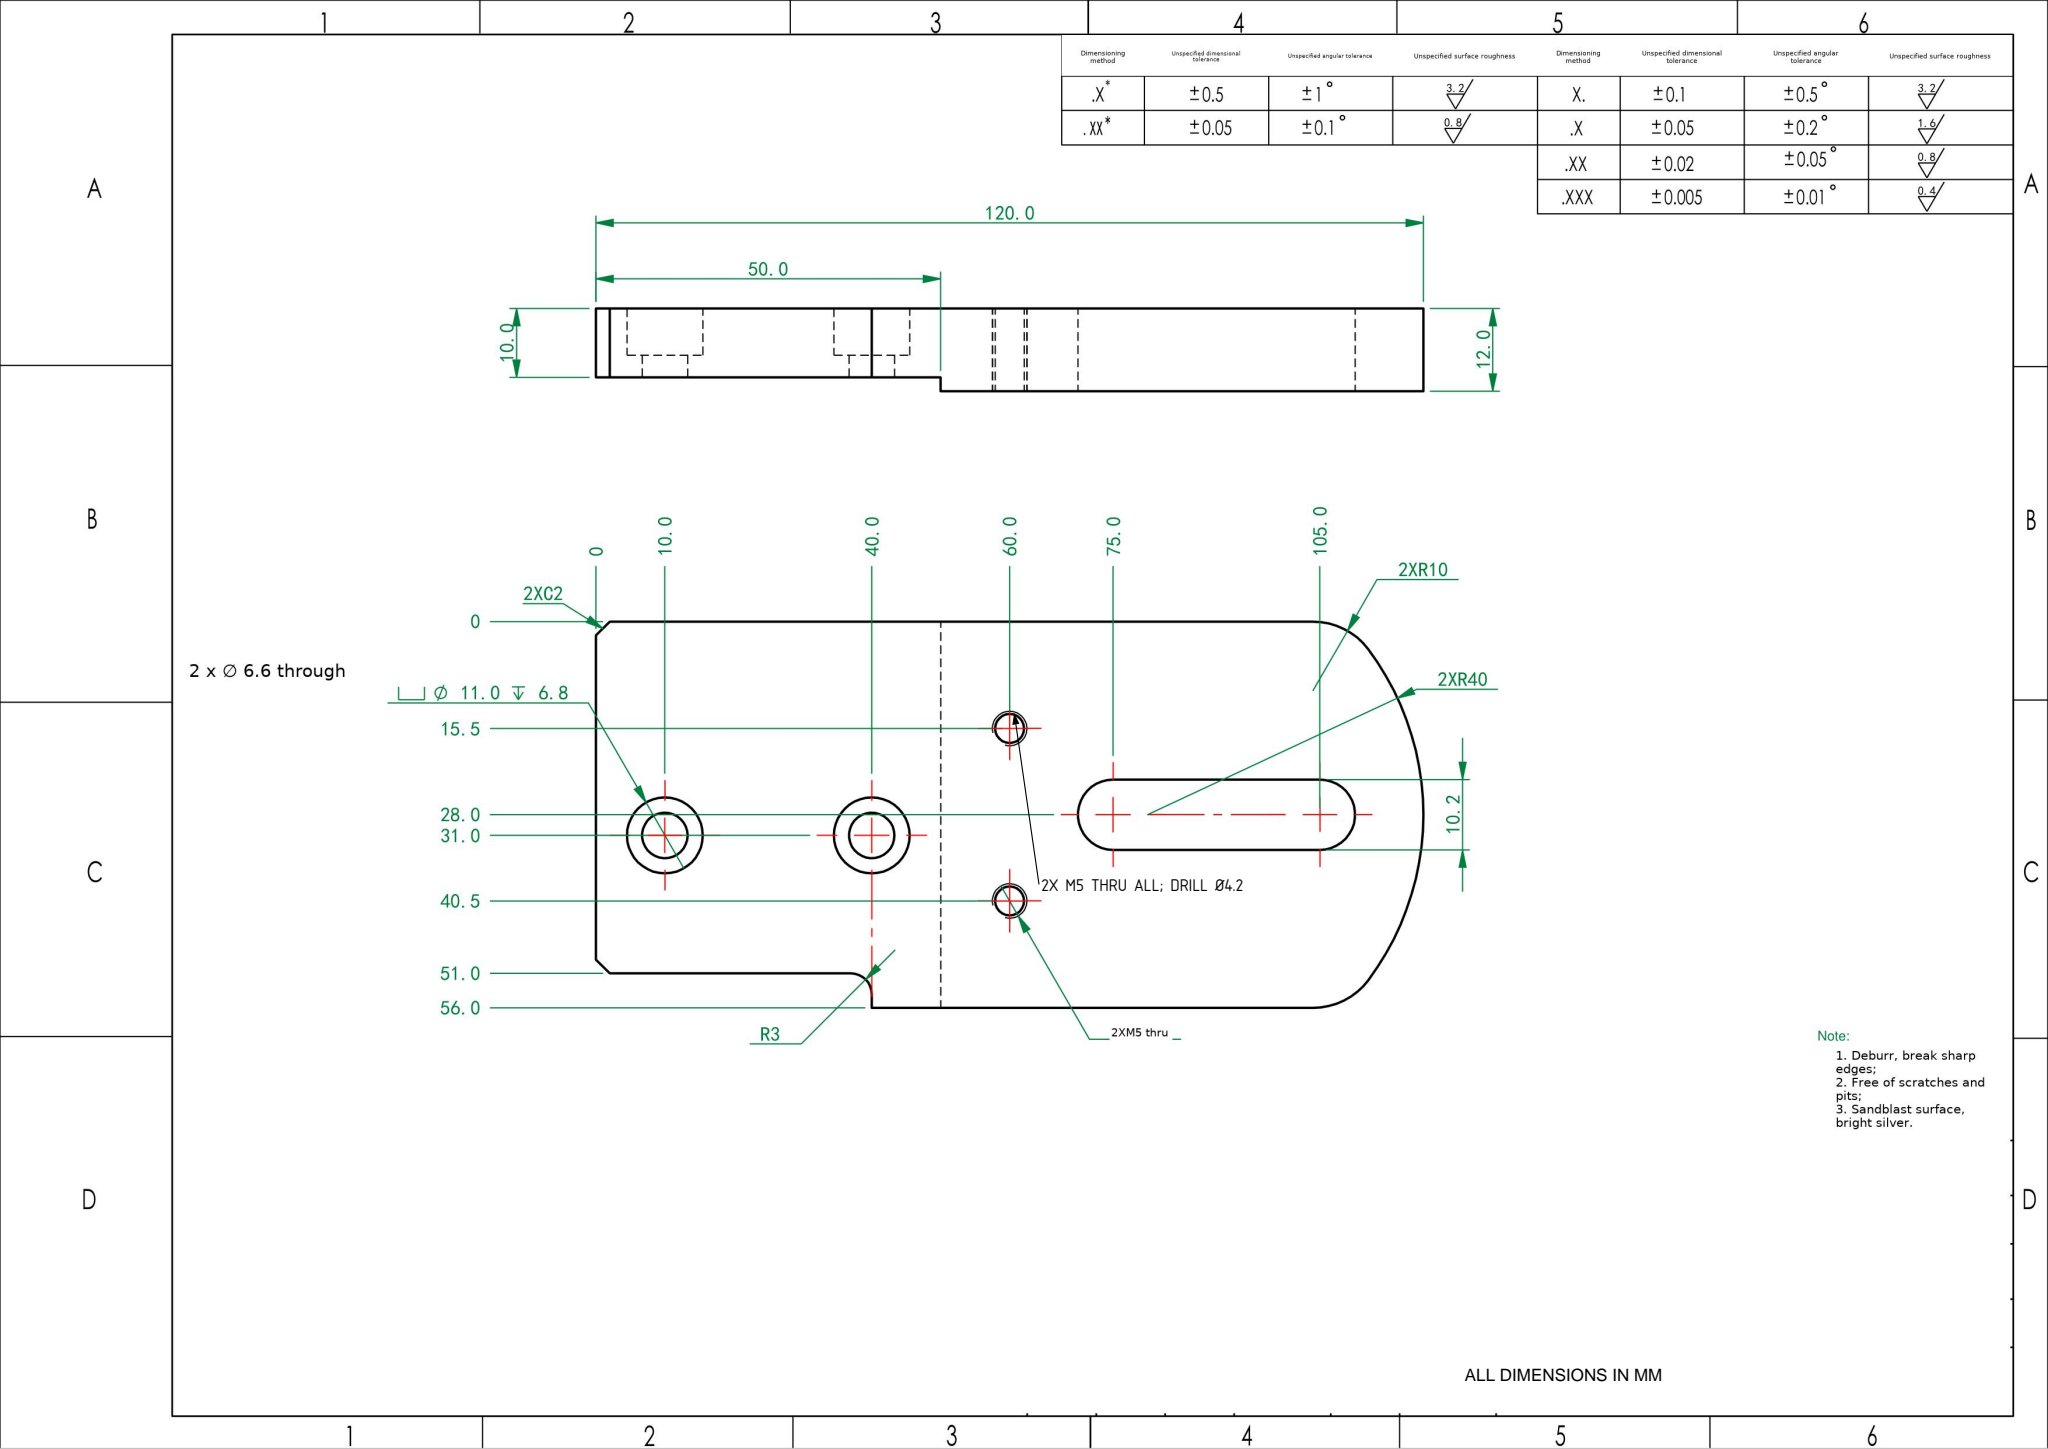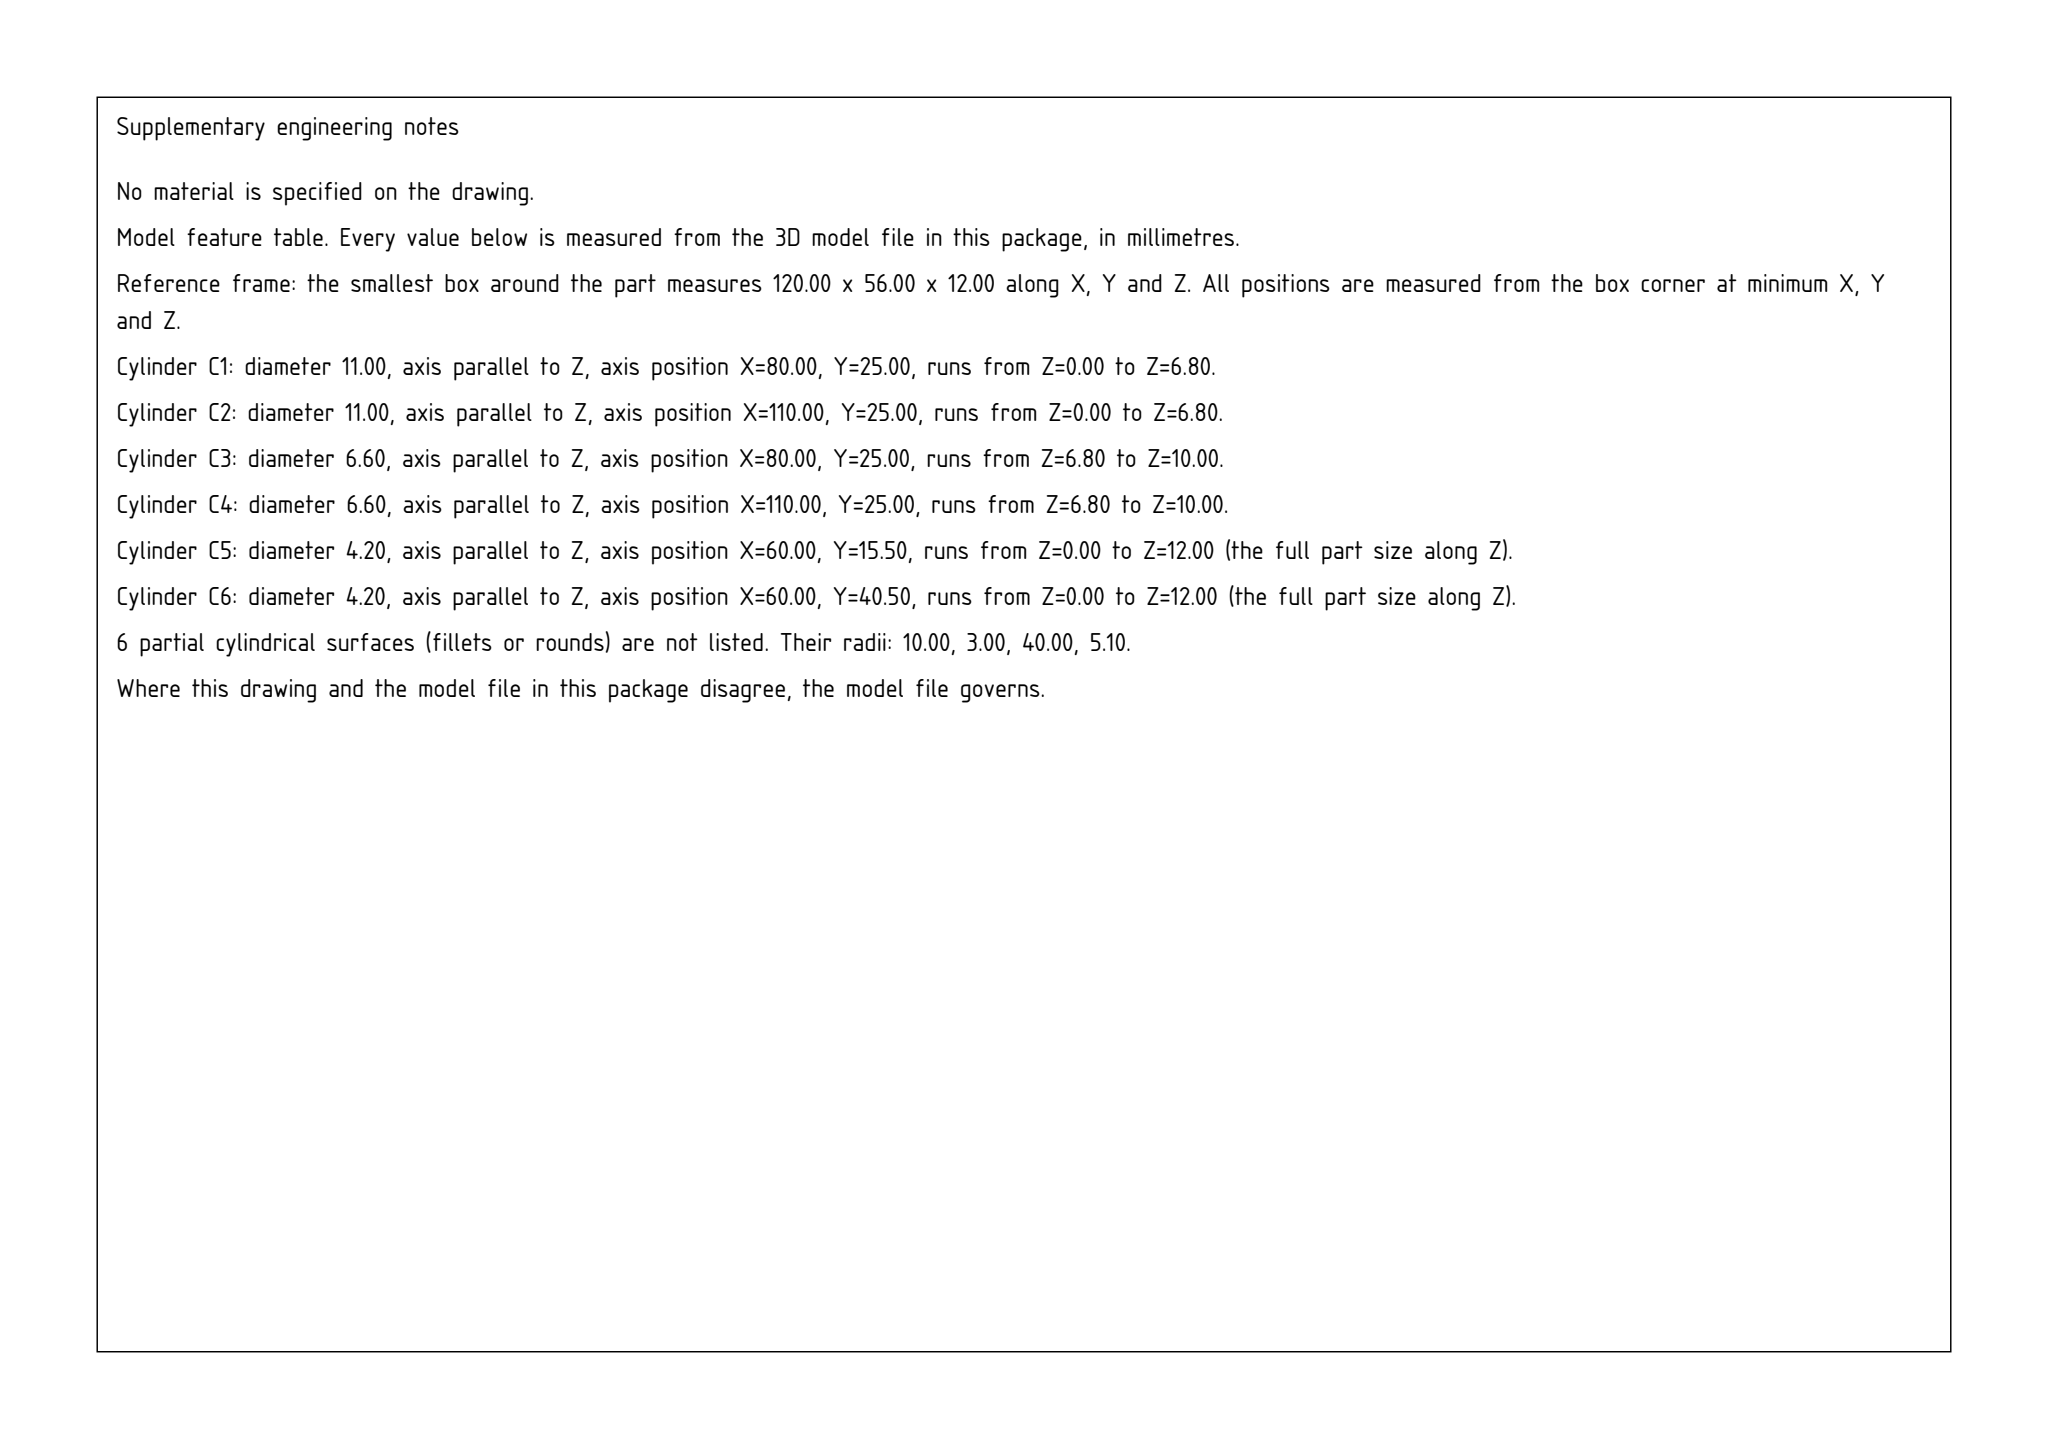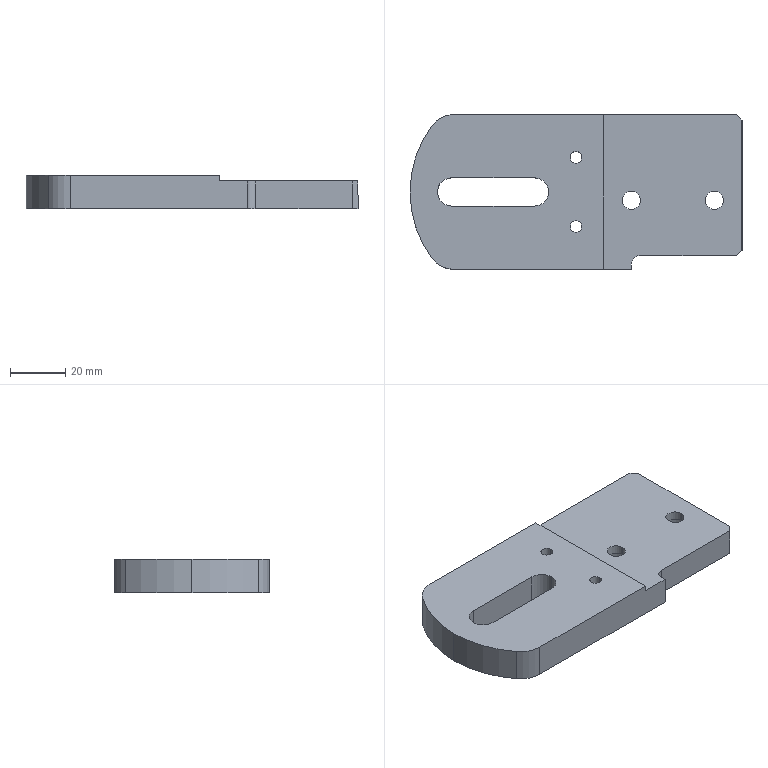Part | SolidWorks | mm | 1 solid | 35 faces | box 120 x 56 x 12 mm | volume 64055 mm3 | cylinder 20 | plane 15 | commonest cylinder face diameters 11 x4 6.6 x4 4.2 x4 10.2 x3 80 x2 20 x2 6 x1
Drawing notes:
2X M5 THRU ALL (12 THK); TAP DRILL Ø4.2 THRU | from the solid: cylinders Ø4.2 z-axis at (60,15.5) & (60,40.5), length 12.0 = full 12.0 plate thickness